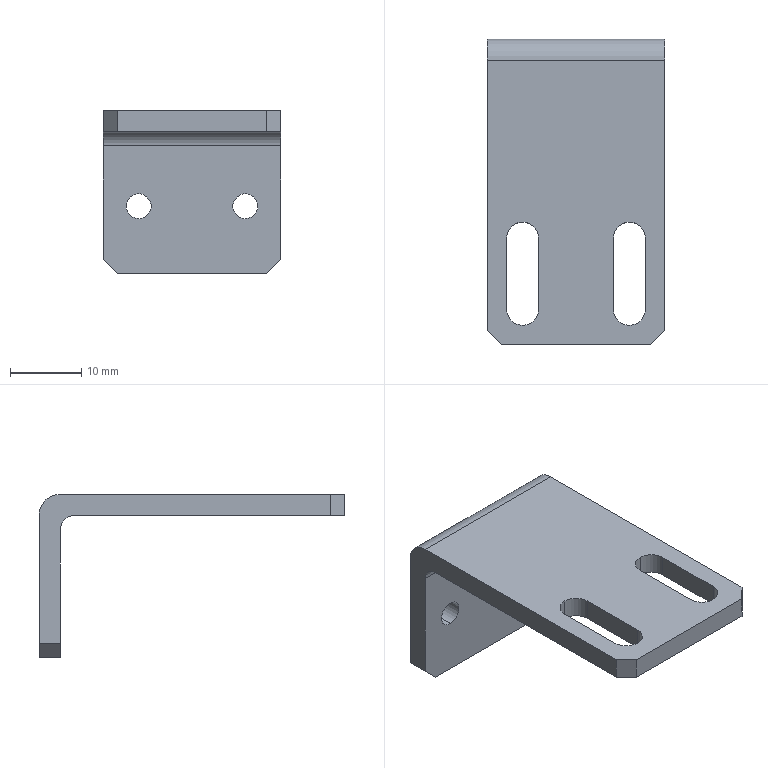Component | SolidWorks | 300-01-1 | 1 solid | 28 faces | box 25 x 43 x 23 mm | volume 4251 mm3 | plane 16 | cylinder 12 | commonest cylinder face diameters 4.5 x6 3.5 x4 6 x1 4 x1 | material SUS304
build123d program:
from build123d import *

# Parameters (mm, degrees)
EXTRUDE_THIN1_DEPTH = 12.5
CUT_EXTRUDE1_DEPTH  = 47.435
SKETCH3_R           = 1.75
CUT_EXTRUDE2_DEPTH  = 50.043
CHAMFER1_SIZE       = 2
FILLET1_R           = 3
FILLET2_R           = 2


with BuildPart() as part:
    # Sketch1 → Extrude-Thin1 (new, symmetric)
    with BuildSketch(Plane(origin=(0, 0, 0), x_dir=(1, 0, 0), z_dir=(0, 1, 0))):
        Polygon((0, 20), (0, 0), (40, 0), (40, -3), (-3, -3), (-3, 20), align=None)
    extrude(amount=EXTRUDE_THIN1_DEPTH, both=True)

    # Sketch2 → Cut-Extrude1 (cut, through all)
    with BuildSketch(Plane(origin=(0, 0, 0), x_dir=(-1, 0, 0), z_dir=(0, 0, -1))):
        with BuildLine():
            Line((-35, 9.75), (-25, 9.75))
            ThreePointArc((-25, 9.75), (-22.75, 7.5), (-25, 5.25))
            Line((-25, 5.25), (-35, 5.25))
            ThreePointArc((-35, 5.25), (-37.25, 7.5), (-35, 9.75))
        make_face()
        with BuildLine():
            Line((-35, -9.75), (-25, -9.75))
            ThreePointArc((-25, -9.75), (-22.75, -7.5), (-25, -5.25))
            Line((-25, -5.25), (-35, -5.25))
            ThreePointArc((-35, -5.25), (-37.25, -7.5), (-35, -9.75))
        make_face()
    extrude(amount=-CUT_EXTRUDE1_DEPTH, mode=Mode.SUBTRACT)

    # Sketch3 → Cut-Extrude2 (cut, through all)
    with BuildSketch(Plane.ZY.offset(3)):
        with Locations((-10.5, 7.5)):
            Circle(SKETCH3_R)
        with Locations((-10.5, -7.5)):
            Circle(SKETCH3_R)
    extrude(amount=-CUT_EXTRUDE2_DEPTH, mode=Mode.SUBTRACT)

    # Chamfer1
    chamfer1_edges = [part.edges().sort_by_distance(p)[0] for p in [
        (-1.5, 12.5, -20),
        (-1.5, -12.5, -20),
        (40, -12.5, 1.5),
        (40, 12.5, 1.5),
    ]]
    chamfer(chamfer1_edges, length=CHAMFER1_SIZE)

    # Fillet1
    fillet1_edges = [part.edges().sort_by_distance(p)[0] for p in [
        (-3, 0, 3),
    ]]
    fillet(fillet1_edges, radius=FILLET1_R)

    # Fillet2
    fillet2_edges = [part.edges().sort_by_distance(p)[0] for p in [
        (0, 0, 0),
    ]]
    fillet(fillet2_edges, radius=FILLET2_R)


solid = part.part

# Placed as in the assembly
solid = solid.moved(Location((230, 175, 115), (0, 0, -90)))
STEP:
#1=CARTESIAN_POINT('',(8.76,6.89,4.183));
#2=VERTEX_POINT('',#1);
#3=CARTESIAN_POINT('',(8.76,6.89,4.045));
#4=VERTEX_POINT('',#3);
#5=CARTESIAN_POINT('',(8.76,6.89,4.114));
#6=DIRECTION('',(-0.,-1.,0.));
#7=DIRECTION('',(0.,0.,-1.));
#8=AXIS2_PLACEMENT_3D('',#5,#6,#7);
#9=CIRCLE('',#8,0.0689);
#10=EDGE_CURVE('',#2,#4,#9,.T.);
#11=ORIENTED_EDGE('',*,*,#10,.T.);
#12=CARTESIAN_POINT('',(8.76,7.008,4.045));
#13=VERTEX_POINT('',#12);
#14=CARTESIAN_POINT('',(8.76,5.315,4.045));
#15=DIRECTION('',(0.,1.,-0.));
#16=VECTOR('',#15,39.37);
#17=LINE('',#14,#16);
#18=EDGE_CURVE('',#4,#13,#17,.T.);
#19=ORIENTED_EDGE('',*,*,#18,.T.);
#20=CARTESIAN_POINT('',(8.76,7.008,4.183));
#21=VERTEX_POINT('',#20);
#22=CARTESIAN_POINT('',(8.76,7.008,4.114));
#23=DIRECTION('',(0.,1.,-0.));
#24=DIRECTION('',(-0.,0.,1.));
#25=AXIS2_PLACEMENT_3D('',#22,#23,#24);
#26=CIRCLE('',#25,0.0689);
#27=EDGE_CURVE('',#13,#21,#26,.T.);
#28=ORIENTED_EDGE('',*,*,#27,.T.);
#29=CARTESIAN_POINT('',(8.76,5.315,4.183));
#30=DIRECTION('',(0.,1.,-0.));
#31=VECTOR('',#30,39.37);
#32=LINE('',#29,#31);
#33=EDGE_CURVE('',#2,#21,#32,.T.);
#34=ORIENTED_EDGE('',*,*,#33,.F.);
#35=EDGE_LOOP('',(#11,#19,#28,#34));
#36=FACE_OUTER_BOUND('',#35,.T.);
#37=CARTESIAN_POINT('',(8.76,5.315,4.114));
#38=DIRECTION('',(0.,1.,-0.));
#39=DIRECTION('',(-0.,0.,1.));
#40=AXIS2_PLACEMENT_3D('',#37,#38,#39);
#41=CYLINDRICAL_SURFACE('',#40,0.0689);
#42=ADVANCED_FACE('',(#36),#41,.F.);
#43=CARTESIAN_POINT('',(9.35,6.89,4.183));
#44=VERTEX_POINT('',#43);
#45=CARTESIAN_POINT('',(9.35,6.89,4.045));
#46=VERTEX_POINT('',#45);
#47=CARTESIAN_POINT('',(9.35,6.89,4.114));
#48=DIRECTION('',(-0.,-1.,0.));
#49=DIRECTION('',(0.,0.,-1.));
#50=AXIS2_PLACEMENT_3D('',#47,#48,#49);
#51=CIRCLE('',#50,0.0689);
#52=EDGE_CURVE('',#44,#46,#51,.T.);
#53=ORIENTED_EDGE('',*,*,#52,.T.);
#54=CARTESIAN_POINT('',(9.35,7.008,4.045));
#55=VERTEX_POINT('',#54);
#56=CARTESIAN_POINT('',(9.35,5.315,4.045));
#57=DIRECTION('',(0.,1.,-0.));
#58=VECTOR('',#57,39.37);
#59=LINE('',#56,#58);
#60=EDGE_CURVE('',#46,#55,#59,.T.);
#61=ORIENTED_EDGE('',*,*,#60,.T.);
#62=CARTESIAN_POINT('',(9.35,7.008,4.183));
#63=VERTEX_POINT('',#62);
#64=CARTESIAN_POINT('',(9.35,7.008,4.114));
#65=DIRECTION('',(0.,1.,-0.));
#66=DIRECTION('',(-0.,0.,1.));
#67=AXIS2_PLACEMENT_3D('',#64,#65,#66);
#68=CIRCLE('',#67,0.0689);
#69=EDGE_CURVE('',#55,#63,#68,.T.);
#70=ORIENTED_EDGE('',*,*,#69,.T.);
#71=CARTESIAN_POINT('',(9.35,5.315,4.183));
#72=DIRECTION('',(0.,1.,-0.));
#73=VECTOR('',#72,39.37);
#74=LINE('',#71,#73);
#75=EDGE_CURVE('',#44,#63,#74,.T.);
#76=ORIENTED_EDGE('',*,*,#75,.F.);
#77=EDGE_LOOP('',(#53,#61,#70,#76));
#78=FACE_OUTER_BOUND('',#77,.T.);
#79=CARTESIAN_POINT('',(9.35,5.315,4.114));
#80=DIRECTION('',(0.,1.,-0.));
#81=DIRECTION('',(-0.,0.,1.));
#82=AXIS2_PLACEMENT_3D('',#79,#80,#81);
#83=CYLINDRICAL_SURFACE('',#82,0.0689);
#84=ADVANCED_FACE('',(#78),#83,.F.);
#85=CARTESIAN_POINT('',(8.76,5.994,4.646));
#86=VERTEX_POINT('',#85);
#87=CARTESIAN_POINT('',(8.848,5.906,4.646));
#88=VERTEX_POINT('',#87);
#89=CARTESIAN_POINT('',(8.76,5.906,4.646));
#90=DIRECTION('',(0.,-0.,-1.));
#91=DIRECTION('',(0.,-1.,0.));
#92=AXIS2_PLACEMENT_3D('',#89,#90,#91);
#93=CIRCLE('',#92,0.08858);
#94=EDGE_CURVE('',#86,#88,#93,.T.);
#95=ORIENTED_EDGE('',*,*,#94,.F.);
#96=CARTESIAN_POINT('',(8.76,5.994,4.528));
#97=VERTEX_POINT('',#96);
#98=CARTESIAN_POINT('',(8.76,5.994,4.646));
#99=DIRECTION('',(0.,-0.,-1.));
#100=VECTOR('',#99,39.37);
#101=LINE('',#98,#100);
#102=EDGE_CURVE('',#86,#97,#101,.T.);
#103=ORIENTED_EDGE('',*,*,#102,.T.);
#104=CARTESIAN_POINT('',(8.848,5.906,4.528));
#105=VERTEX_POINT('',#104);
#106=CARTESIAN_POINT('',(8.76,5.906,4.528));
#107=DIRECTION('',(0.,-0.,-1.));
#108=DIRECTION('',(0.,-1.,0.));
#109=AXIS2_PLACEMENT_3D('',#106,#107,#108);
#110=CIRCLE('',#109,0.08858);
#111=EDGE_CURVE('',#97,#105,#110,.T.);
#112=ORIENTED_EDGE('',*,*,#111,.T.);
#113=CARTESIAN_POINT('',(8.848,5.906,4.646));
#114=DIRECTION('',(0.,-0.,-1.));
#115=VECTOR('',#114,39.37);
#116=LINE('',#113,#115);
#117=EDGE_CURVE('',#88,#105,#116,.T.);
#118=ORIENTED_EDGE('',*,*,#117,.F.);
#119=EDGE_LOOP('',(#95,#103,#112,#118));
#120=FACE_OUTER_BOUND('',#119,.T.);
#121=CARTESIAN_POINT('',(8.76,5.906,4.646));
#122=DIRECTION('',(0.,-0.,-1.));
#123=DIRECTION('',(0.,1.,0.));
#124=AXIS2_PLACEMENT_3D('',#121,#122,#123);
#125=CYLINDRICAL_SURFACE('',#124,0.08858);
#126=ADVANCED_FACE('',(#120),#125,.F.);
#127=CARTESIAN_POINT('',(9.35,5.994,4.646));
#128=VERTEX_POINT('',#127);
#129=CARTESIAN_POINT('',(9.439,5.906,4.646));
#130=VERTEX_POINT('',#129);
#131=CARTESIAN_POINT('',(9.35,5.906,4.646));
#132=DIRECTION('',(0.,-0.,-1.));
#133=DIRECTION('',(0.,1.,0.));
#134=AXIS2_PLACEMENT_3D('',#131,#132,#133);
#135=CIRCLE('',#134,0.08858);
#136=EDGE_CURVE('',#128,#130,#135,.T.);
#137=ORIENTED_EDGE('',*,*,#136,.F.);
#138=CARTESIAN_POINT('',(9.35,5.994,4.528));
#139=VERTEX_POINT('',#138);
#140=CARTESIAN_POINT('',(9.35,5.994,4.646));
#141=DIRECTION('',(0.,-0.,-1.));
#142=VECTOR('',#141,39.37);
#143=LINE('',#140,#142);
#144=EDGE_CURVE('',#128,#139,#143,.T.);
#145=ORIENTED_EDGE('',*,*,#144,.T.);
#146=CARTESIAN_POINT('',(9.439,5.906,4.528));
#147=VERTEX_POINT('',#146);
#148=CARTESIAN_POINT('',(9.35,5.906,4.528));
#149=DIRECTION('',(0.,-0.,-1.));
#150=DIRECTION('',(0.,1.,0.));
#151=AXIS2_PLACEMENT_3D('',#148,#149,#150);
#152=CIRCLE('',#151,0.08858);
#153=EDGE_CURVE('',#139,#147,#152,.T.);
#154=ORIENTED_EDGE('',*,*,#153,.T.);
#155=CARTESIAN_POINT('',(9.439,5.906,4.646));
#156=DIRECTION('',(0.,-0.,-1.));
#157=VECTOR('',#156,39.37);
#158=LINE('',#155,#157);
#159=EDGE_CURVE('',#130,#147,#158,.T.);
#160=ORIENTED_EDGE('',*,*,#159,.F.);
#161=EDGE_LOOP('',(#137,#145,#154,#160));
#162=FACE_OUTER_BOUND('',#161,.T.);
#163=CARTESIAN_POINT('',(9.35,5.906,4.646));
#164=DIRECTION('',(0.,-0.,-1.));
#165=DIRECTION('',(0.,1.,0.));
#166=AXIS2_PLACEMENT_3D('',#163,#164,#165);
#167=CYLINDRICAL_SURFACE('',#166,0.08858);
#168=ADVANCED_FACE('',(#162),#167,.F.);
#169=CARTESIAN_POINT('',(8.848,5.512,4.646));
#170=VERTEX_POINT('',#169);
#171=CARTESIAN_POINT('',(8.848,5.512,4.646));
#172=DIRECTION('',(-0.,-1.,0.));
#173=VECTOR('',#172,39.37);
#174=LINE('',#171,#173);
#175=EDGE_CURVE('',#88,#170,#174,.T.);
#176=ORIENTED_EDGE('',*,*,#175,.T.);
#177=CARTESIAN_POINT('',(8.671,5.512,4.646));
#178=VERTEX_POINT('',#177);
#179=CARTESIAN_POINT('',(8.76,5.512,4.646));
#180=DIRECTION('',(0.,-0.,-1.));
#181=DIRECTION('',(0.,-1.,0.));
#182=AXIS2_PLACEMENT_3D('',#179,#180,#181);
#183=CIRCLE('',#182,0.08858);
#184=EDGE_CURVE('',#170,#178,#183,.T.);
#185=ORIENTED_EDGE('',*,*,#184,.T.);
#186=CARTESIAN_POINT('',(8.671,5.906,4.646));
#187=VERTEX_POINT('',#186);
#188=CARTESIAN_POINT('',(8.671,5.512,4.646));
#189=DIRECTION('',(0.,1.,-0.));
#190=VECTOR('',#189,39.37);
#191=LINE('',#188,#190);
#192=EDGE_CURVE('',#178,#187,#191,.T.);
#193=ORIENTED_EDGE('',*,*,#192,.T.);
#194=CARTESIAN_POINT('',(8.76,5.906,4.646));
#195=DIRECTION('',(0.,-0.,-1.));
#196=DIRECTION('',(0.,-1.,0.));
#197=AXIS2_PLACEMENT_3D('',#194,#195,#196);
#198=CIRCLE('',#197,0.08858);
#199=EDGE_CURVE('',#187,#86,#198,.T.);
#200=ORIENTED_EDGE('',*,*,#199,.T.);
#201=ORIENTED_EDGE('',*,*,#94,.T.);
#202=EDGE_LOOP('',(#176,#185,#193,#200,#201));
#203=FACE_BOUND('',#202,.T.);
#204=CARTESIAN_POINT('',(9.439,5.512,4.646));
#205=VERTEX_POINT('',#204);
#206=CARTESIAN_POINT('',(9.439,5.512,4.646));
#207=DIRECTION('',(0.,-1.,0.));
#208=VECTOR('',#207,39.37);
#209=LINE('',#206,#208);
#210=EDGE_CURVE('',#130,#205,#209,.T.);
#211=ORIENTED_EDGE('',*,*,#210,.T.);
#212=CARTESIAN_POINT('',(9.262,5.512,4.646));
#213=VERTEX_POINT('',#212);
#214=CARTESIAN_POINT('',(9.35,5.512,4.646));
#215=DIRECTION('',(0.,-0.,-1.));
#216=DIRECTION('',(0.,1.,0.));
#217=AXIS2_PLACEMENT_3D('',#214,#215,#216);
#218=CIRCLE('',#217,0.08858);
#219=EDGE_CURVE('',#205,#213,#218,.T.);
#220=ORIENTED_EDGE('',*,*,#219,.T.);
#221=CARTESIAN_POINT('',(9.262,5.906,4.646));
#222=VERTEX_POINT('',#221);
#223=CARTESIAN_POINT('',(9.262,5.512,4.646));
#224=DIRECTION('',(0.,1.,-0.));
#225=VECTOR('',#224,39.37);
#226=LINE('',#223,#225);
#227=EDGE_CURVE('',#213,#222,#226,.T.);
#228=ORIENTED_EDGE('',*,*,#227,.T.);
#229=CARTESIAN_POINT('',(9.35,5.906,4.646));
#230=DIRECTION('',(0.,-0.,-1.));
#231=DIRECTION('',(0.,1.,0.));
#232=AXIS2_PLACEMENT_3D('',#229,#230,#231);
#233=CIRCLE('',#232,0.08858);
#234=EDGE_CURVE('',#222,#128,#233,.T.);
#235=ORIENTED_EDGE('',*,*,#234,.T.);
#236=ORIENTED_EDGE('',*,*,#136,.T.);
#237=EDGE_LOOP('',(#211,#220,#228,#235,#236));
#238=FACE_BOUND('',#237,.T.);
#239=CARTESIAN_POINT('',(9.547,6.89,4.646));
#240=VERTEX_POINT('',#239);
#241=CARTESIAN_POINT('',(9.547,5.394,4.646));
#242=VERTEX_POINT('',#241);
#243=CARTESIAN_POINT('',(9.547,6.89,4.646));
#244=DIRECTION('',(-0.,-1.,0.));
#245=VECTOR('',#244,39.37);
#246=LINE('',#243,#245);
#247=EDGE_CURVE('',#240,#242,#246,.T.);
#248=ORIENTED_EDGE('',*,*,#247,.F.);
#249=CARTESIAN_POINT('',(8.563,6.89,4.646));
#250=VERTEX_POINT('',#249);
#251=CARTESIAN_POINT('',(9.547,6.89,4.646));
#252=DIRECTION('',(-1.,0.,-0.));
#253=VECTOR('',#252,39.37);
#254=LINE('',#251,#253);
#255=EDGE_CURVE('',#240,#250,#254,.T.);
#256=ORIENTED_EDGE('',*,*,#255,.T.);
#257=CARTESIAN_POINT('',(8.563,5.394,4.646));
#258=VERTEX_POINT('',#257);
#259=CARTESIAN_POINT('',(8.563,6.89,4.646));
#260=DIRECTION('',(-0.,-1.,0.));
#261=VECTOR('',#260,39.37);
#262=LINE('',#259,#261);
#263=EDGE_CURVE('',#250,#258,#262,.T.);
#264=ORIENTED_EDGE('',*,*,#263,.T.);
#265=CARTESIAN_POINT('',(8.642,5.315,4.646));
#266=VERTEX_POINT('',#265);
#267=CARTESIAN_POINT('',(8.563,5.394,4.646));
#268=DIRECTION('',(0.7071,-0.7071,0.));
#269=VECTOR('',#268,39.37);
#270=LINE('',#267,#269);
#271=EDGE_CURVE('',#258,#266,#270,.T.);
#272=ORIENTED_EDGE('',*,*,#271,.T.);
#273=CARTESIAN_POINT('',(9.469,5.315,4.646));
#274=VERTEX_POINT('',#273);
#275=CARTESIAN_POINT('',(9.547,5.315,4.646));
#276=DIRECTION('',(-1.,0.,-0.));
#277=VECTOR('',#276,39.37);
#278=LINE('',#275,#277);
#279=EDGE_CURVE('',#274,#266,#278,.T.);
#280=ORIENTED_EDGE('',*,*,#279,.F.);
#281=CARTESIAN_POINT('',(9.469,5.315,4.646));
#282=DIRECTION('',(0.7071,0.7071,0.));
#283=VECTOR('',#282,39.37);
#284=LINE('',#281,#283);
#285=EDGE_CURVE('',#274,#242,#284,.T.);
#286=ORIENTED_EDGE('',*,*,#285,.T.);
#287=EDGE_LOOP('',(#248,#256,#264,#272,#280,#286));
#288=FACE_OUTER_BOUND('',#287,.T.);
#289=CARTESIAN_POINT('',(9.547,6.89,4.646));
#290=DIRECTION('',(0.,-0.,-1.));
#291=DIRECTION('',(0.,1.,-0.));
#292=AXIS2_PLACEMENT_3D('',#289,#290,#291);
#293=PLANE('',#292);
#294=ADVANCED_FACE('',(#203,#238,#288),#293,.F.);
#295=CARTESIAN_POINT('',(9.469,5.315,4.528));
#296=VERTEX_POINT('',#295);
#297=CARTESIAN_POINT('',(8.642,5.315,4.528));
#298=VERTEX_POINT('',#297);
#299=CARTESIAN_POINT('',(9.547,5.315,4.528));
#300=DIRECTION('',(-1.,0.,-0.));
#301=VECTOR('',#300,39.37);
#302=LINE('',#299,#301);
#303=EDGE_CURVE('',#296,#298,#302,.T.);
#304=ORIENTED_EDGE('',*,*,#303,.F.);
#305=CARTESIAN_POINT('',(9.469,5.315,4.646));
#306=DIRECTION('',(-0.,0.,1.));
#307=VECTOR('',#306,39.37);
#308=LINE('',#305,#307);
#309=EDGE_CURVE('',#296,#274,#308,.T.);
#310=ORIENTED_EDGE('',*,*,#309,.T.);
#311=ORIENTED_EDGE('',*,*,#279,.T.);
#312=CARTESIAN_POINT('',(8.642,5.315,4.528));
#313=DIRECTION('',(0.,-0.,-1.));
#314=VECTOR('',#313,39.37);
#315=LINE('',#312,#314);
#316=EDGE_CURVE('',#266,#298,#315,.T.);
#317=ORIENTED_EDGE('',*,*,#316,.T.);
#318=EDGE_LOOP('',(#304,#310,#311,#317));
#319=FACE_OUTER_BOUND('',#318,.T.);
#320=CARTESIAN_POINT('',(9.547,5.315,4.528));
#321=DIRECTION('',(-0.,-1.,0.));
#322=DIRECTION('',(0.,-0.,-1.));
#323=AXIS2_PLACEMENT_3D('',#320,#321,#322);
#324=PLANE('',#323);
#325=ADVANCED_FACE('',(#319),#324,.T.);
#326=CARTESIAN_POINT('',(8.848,5.512,4.528));
#327=VERTEX_POINT('',#326);
#328=CARTESIAN_POINT('',(8.671,5.512,4.528));
#329=VERTEX_POINT('',#328);
#330=CARTESIAN_POINT('',(8.76,5.512,4.528));
#331=DIRECTION('',(0.,-0.,-1.));
#332=DIRECTION('',(0.,-1.,0.));
#333=AXIS2_PLACEMENT_3D('',#330,#331,#332);
#334=CIRCLE('',#333,0.08858);
#335=EDGE_CURVE('',#327,#329,#334,.T.);
#336=ORIENTED_EDGE('',*,*,#335,.F.);
#337=CARTESIAN_POINT('',(8.848,5.512,4.528));
#338=DIRECTION('',(-0.,-1.,0.));
#339=VECTOR('',#338,39.37);
#340=LINE('',#337,#339);
#341=EDGE_CURVE('',#105,#327,#340,.T.);
#342=ORIENTED_EDGE('',*,*,#341,.F.);
#343=ORIENTED_EDGE('',*,*,#111,.F.);
#344=CARTESIAN_POINT('',(8.671,5.906,4.528));
#345=VERTEX_POINT('',#344);
#346=CARTESIAN_POINT('',(8.76,5.906,4.528));
#347=DIRECTION('',(0.,-0.,-1.));
#348=DIRECTION('',(0.,-1.,0.));
#349=AXIS2_PLACEMENT_3D('',#346,#347,#348);
#350=CIRCLE('',#349,0.08858);
#351=EDGE_CURVE('',#345,#97,#350,.T.);
#352=ORIENTED_EDGE('',*,*,#351,.F.);
#353=CARTESIAN_POINT('',(8.671,5.512,4.528));
#354=DIRECTION('',(0.,1.,-0.));
#355=VECTOR('',#354,39.37);
#356=LINE('',#353,#355);
#357=EDGE_CURVE('',#329,#345,#356,.T.);
#358=ORIENTED_EDGE('',*,*,#357,.F.);
#359=EDGE_LOOP('',(#336,#342,#343,#352,#358));
#360=FACE_BOUND('',#359,.T.);
#361=CARTESIAN_POINT('',(9.439,5.512,4.528));
#362=VERTEX_POINT('',#361);
#363=CARTESIAN_POINT('',(9.262,5.512,4.528));
#364=VERTEX_POINT('',#363);
#365=CARTESIAN_POINT('',(9.35,5.512,4.528));
#366=DIRECTION('',(0.,-0.,-1.));
#367=DIRECTION('',(0.,1.,0.));
#368=AXIS2_PLACEMENT_3D('',#365,#366,#367);
#369=CIRCLE('',#368,0.08858);
#370=EDGE_CURVE('',#362,#364,#369,.T.);
#371=ORIENTED_EDGE('',*,*,#370,.F.);
#372=CARTESIAN_POINT('',(9.439,5.512,4.528));
#373=DIRECTION('',(0.,-1.,0.));
#374=VECTOR('',#373,39.37);
#375=LINE('',#372,#374);
#376=EDGE_CURVE('',#147,#362,#375,.T.);
#377=ORIENTED_EDGE('',*,*,#376,.F.);
#378=ORIENTED_EDGE('',*,*,#153,.F.);
#379=CARTESIAN_POINT('',(9.262,5.906,4.528));
#380=VERTEX_POINT('',#379);
#381=CARTESIAN_POINT('',(9.35,5.906,4.528));
#382=DIRECTION('',(0.,-0.,-1.));
#383=DIRECTION('',(0.,1.,0.));
#384=AXIS2_PLACEMENT_3D('',#381,#382,#383);
#385=CIRCLE('',#384,0.08858);
#386=EDGE_CURVE('',#380,#139,#385,.T.);
#387=ORIENTED_EDGE('',*,*,#386,.F.);
#388=CARTESIAN_POINT('',(9.262,5.512,4.528));
#389=DIRECTION('',(0.,1.,-0.));
#390=VECTOR('',#389,39.37);
#391=LINE('',#388,#390);
#392=EDGE_CURVE('',#364,#380,#391,.T.);
#393=ORIENTED_EDGE('',*,*,#392,.F.);
#394=EDGE_LOOP('',(#371,#377,#378,#387,#393));
#395=FACE_BOUND('',#394,.T.);
#396=CARTESIAN_POINT('',(8.563,6.811,4.528));
#397=VERTEX_POINT('',#396);
#398=CARTESIAN_POINT('',(8.563,5.394,4.528));
#399=VERTEX_POINT('',#398);
#400=CARTESIAN_POINT('',(8.563,6.89,4.528));
#401=DIRECTION('',(-0.,-1.,0.));
#402=VECTOR('',#401,39.37);
#403=LINE('',#400,#402);
#404=EDGE_CURVE('',#397,#399,#403,.T.);
#405=ORIENTED_EDGE('',*,*,#404,.F.);
#406=CARTESIAN_POINT('',(9.547,6.811,4.528));
#407=VERTEX_POINT('',#406);
#408=CARTESIAN_POINT('',(9.547,6.811,4.528));
#409=DIRECTION('',(1.,-0.,0.));
#410=VECTOR('',#409,39.37);
#411=LINE('',#408,#410);
#412=EDGE_CURVE('',#397,#407,#411,.T.);
#413=ORIENTED_EDGE('',*,*,#412,.T.);
#414=CARTESIAN_POINT('',(9.547,5.394,4.528));
#415=VERTEX_POINT('',#414);
#416=CARTESIAN_POINT('',(9.547,6.89,4.528));
#417=DIRECTION('',(-0.,-1.,0.));
#418=VECTOR('',#417,39.37);
#419=LINE('',#416,#418);
#420=EDGE_CURVE('',#407,#415,#419,.T.);
#421=ORIENTED_EDGE('',*,*,#420,.T.);
#422=CARTESIAN_POINT('',(10.295,6.142,4.528));
#423=DIRECTION('',(-0.7071,-0.7071,-0.));
#424=VECTOR('',#423,39.37);
#425=LINE('',#422,#424);
#426=EDGE_CURVE('',#415,#296,#425,.T.);
#427=ORIENTED_EDGE('',*,*,#426,.T.);
#428=ORIENTED_EDGE('',*,*,#303,.T.);
#429=CARTESIAN_POINT('',(8.307,5.65,4.528));
#430=DIRECTION('',(-0.7071,0.7071,-0.));
#431=VECTOR('',#430,39.37);
#432=LINE('',#429,#431);
#433=EDGE_CURVE('',#298,#399,#432,.T.);
#434=ORIENTED_EDGE('',*,*,#433,.T.);
#435=EDGE_LOOP('',(#405,#413,#421,#427,#428,#434));
#436=FACE_OUTER_BOUND('',#435,.T.);
#437=CARTESIAN_POINT('',(9.547,6.89,4.528));
#438=DIRECTION('',(0.,-0.,-1.));
#439=DIRECTION('',(0.,1.,-0.));
#440=AXIS2_PLACEMENT_3D('',#437,#438,#439);
#441=PLANE('',#440);
#442=ADVANCED_FACE('',(#360,#395,#436),#441,.T.);
#443=ORIENTED_EDGE('',*,*,#10,.F.);
#444=CARTESIAN_POINT('',(8.76,6.89,4.114));
#445=DIRECTION('',(-0.,-1.,0.));
#446=DIRECTION('',(0.,0.,-1.));
#447=AXIS2_PLACEMENT_3D('',#444,#445,#446);
#448=CIRCLE('',#447,0.0689);
#449=EDGE_CURVE('',#4,#2,#448,.T.);
#450=ORIENTED_EDGE('',*,*,#449,.F.);
#451=EDGE_LOOP('',(#443,#450));
#452=FACE_BOUND('',#451,.T.);
#453=ORIENTED_EDGE('',*,*,#52,.F.);
#454=CARTESIAN_POINT('',(9.35,6.89,4.114));
#455=DIRECTION('',(-0.,-1.,0.));
#456=DIRECTION('',(0.,0.,-1.));
#457=AXIS2_PLACEMENT_3D('',#454,#455,#456);
#458=CIRCLE('',#457,0.0689);
#459=EDGE_CURVE('',#46,#44,#458,.T.);
#460=ORIENTED_EDGE('',*,*,#459,.F.);
#461=EDGE_LOOP('',(#453,#460));
#462=FACE_BOUND('',#461,.T.);
#463=CARTESIAN_POINT('',(9.547,6.89,3.819));
#464=VERTEX_POINT('',#463);
#465=CARTESIAN_POINT('',(9.547,6.89,4.449));
#466=VERTEX_POINT('',#465);
#467=CARTESIAN_POINT('',(9.547,6.89,3.74));
#468=DIRECTION('',(-0.,0.,1.));
#469=VECTOR('',#468,39.37);
#470=LINE('',#467,#469);
#471=EDGE_CURVE('',#464,#466,#470,.T.);
#472=ORIENTED_EDGE('',*,*,#471,.T.);
#473=CARTESIAN_POINT('',(8.563,6.89,4.449));
#474=VERTEX_POINT('',#473);
#475=CARTESIAN_POINT('',(8.563,6.89,4.449));
#476=DIRECTION('',(-1.,0.,-0.));
#477=VECTOR('',#476,39.37);
#478=LINE('',#475,#477);
#479=EDGE_CURVE('',#466,#474,#478,.T.);
#480=ORIENTED_EDGE('',*,*,#479,.T.);
#481=CARTESIAN_POINT('',(8.563,6.89,3.819));
#482=VERTEX_POINT('',#481);
#483=CARTESIAN_POINT('',(8.563,6.89,3.74));
#484=DIRECTION('',(-0.,0.,1.));
#485=VECTOR('',#484,39.37);
#486=LINE('',#483,#485);
#487=EDGE_CURVE('',#482,#474,#486,.T.);
#488=ORIENTED_EDGE('',*,*,#487,.F.);
#489=CARTESIAN_POINT('',(8.642,6.89,3.74));
#490=VERTEX_POINT('',#489);
#491=CARTESIAN_POINT('',(9.094,6.89,3.287));
#492=DIRECTION('',(0.7071,-0.,-0.7071));
#493=VECTOR('',#492,39.37);
#494=LINE('',#491,#493);
#495=EDGE_CURVE('',#482,#490,#494,.T.);
#496=ORIENTED_EDGE('',*,*,#495,.T.);
#497=CARTESIAN_POINT('',(9.469,6.89,3.74));
#498=VERTEX_POINT('',#497);
#499=CARTESIAN_POINT('',(9.547,6.89,3.74));
#500=DIRECTION('',(-1.,0.,-0.));
#501=VECTOR('',#500,39.37);
#502=LINE('',#499,#501);
#503=EDGE_CURVE('',#498,#490,#502,.T.);
#504=ORIENTED_EDGE('',*,*,#503,.F.);
#505=CARTESIAN_POINT('',(9.508,6.89,3.78));
#506=DIRECTION('',(0.7071,0.,0.7071));
#507=VECTOR('',#506,39.37);
#508=LINE('',#505,#507);
#509=EDGE_CURVE('',#498,#464,#508,.T.);
#510=ORIENTED_EDGE('',*,*,#509,.T.);
#511=EDGE_LOOP('',(#472,#480,#488,#496,#504,#510));
#512=FACE_OUTER_BOUND('',#511,.T.);
#513=CARTESIAN_POINT('',(9.547,6.89,3.74));
#514=DIRECTION('',(-0.,-1.,0.));
#515=DIRECTION('',(0.,-0.,-1.));
#516=AXIS2_PLACEMENT_3D('',#513,#514,#515);
#517=PLANE('',#516);
#518=ADVANCED_FACE('',(#452,#462,#512),#517,.T.);
#519=ORIENTED_EDGE('',*,*,#503,.T.);
#520=CARTESIAN_POINT('',(8.642,7.008,3.74));
#521=VERTEX_POINT('',#520);
#522=CARTESIAN_POINT('',(8.642,7.008,3.74));
#523=DIRECTION('',(0.,1.,-0.));
#524=VECTOR('',#523,39.37);
#525=LINE('',#522,#524);
#526=EDGE_CURVE('',#490,#521,#525,.T.);
#527=ORIENTED_EDGE('',*,*,#526,.T.);
#528=CARTESIAN_POINT('',(9.469,7.008,3.74));
#529=VERTEX_POINT('',#528);
#530=CARTESIAN_POINT('',(9.547,7.008,3.74));
#531=DIRECTION('',(-1.,0.,-0.));
#532=VECTOR('',#531,39.37);
#533=LINE('',#530,#532);
#534=EDGE_CURVE('',#529,#521,#533,.T.);
#535=ORIENTED_EDGE('',*,*,#534,.F.);
#536=CARTESIAN_POINT('',(9.469,6.89,3.74));
#537=DIRECTION('',(-0.,-1.,0.));
#538=VECTOR('',#537,39.37);
#539=LINE('',#536,#538);
#540=EDGE_CURVE('',#529,#498,#539,.T.);
#541=ORIENTED_EDGE('',*,*,#540,.T.);
#542=EDGE_LOOP('',(#519,#527,#535,#541));
#543=FACE_OUTER_BOUND('',#542,.T.);
#544=CARTESIAN_POINT('',(9.547,7.008,3.74));
#545=DIRECTION('',(0.,-0.,-1.));
#546=DIRECTION('',(0.,1.,-0.));
#547=AXIS2_PLACEMENT_3D('',#544,#545,#546);
#548=PLANE('',#547);
#549=ADVANCED_FACE('',(#543),#548,.T.);
#550=CARTESIAN_POINT('',(8.76,7.008,4.114));
#551=DIRECTION('',(0.,1.,-0.));
#552=DIRECTION('',(-0.,0.,1.));
#553=AXIS2_PLACEMENT_3D('',#550,#551,#552);
#554=CIRCLE('',#553,0.0689);
#555=EDGE_CURVE('',#21,#13,#554,.T.);
#556=ORIENTED_EDGE('',*,*,#555,.F.);
#557=ORIENTED_EDGE('',*,*,#27,.F.);
#558=EDGE_LOOP('',(#556,#557));
#559=FACE_BOUND('',#558,.T.);
#560=CARTESIAN_POINT('',(9.35,7.008,4.114));
#561=DIRECTION('',(0.,1.,-0.));
#562=DIRECTION('',(-0.,0.,1.));
#563=AXIS2_PLACEMENT_3D('',#560,#561,#562);
#564=CIRCLE('',#563,0.0689);
#565=EDGE_CURVE('',#63,#55,#564,.T.);
#566=ORIENTED_EDGE('',*,*,#565,.F.);
#567=ORIENTED_EDGE('',*,*,#69,.F.);
#568=EDGE_LOOP('',(#566,#567));
#569=FACE_BOUND('',#568,.T.);
#570=CARTESIAN_POINT('',(8.563,7.008,3.819));
#571=VERTEX_POINT('',#570);
#572=CARTESIAN_POINT('',(8.563,7.008,4.528));
#573=VERTEX_POINT('',#572);
#574=CARTESIAN_POINT('',(8.563,7.008,3.74));
#575=DIRECTION('',(-0.,0.,1.));
#576=VECTOR('',#575,39.37);
#577=LINE('',#574,#576);
#578=EDGE_CURVE('',#571,#573,#577,.T.);
#579=ORIENTED_EDGE('',*,*,#578,.T.);
#580=CARTESIAN_POINT('',(9.547,7.008,4.528));
#581=VERTEX_POINT('',#580);
#582=CARTESIAN_POINT('',(9.547,7.008,4.528));
#583=DIRECTION('',(1.,-0.,0.));
#584=VECTOR('',#583,39.37);
#585=LINE('',#582,#584);
#586=EDGE_CURVE('',#573,#581,#585,.T.);
#587=ORIENTED_EDGE('',*,*,#586,.T.);
#588=CARTESIAN_POINT('',(9.547,7.008,3.819));
#589=VERTEX_POINT('',#588);
#590=CARTESIAN_POINT('',(9.547,7.008,3.74));
#591=DIRECTION('',(-0.,0.,1.));
#592=VECTOR('',#591,39.37);
#593=LINE('',#590,#592);
#594=EDGE_CURVE('',#589,#581,#593,.T.);
#595=ORIENTED_EDGE('',*,*,#594,.F.);
#596=CARTESIAN_POINT('',(9.469,7.008,3.74));
#597=DIRECTION('',(-0.7071,-0.,-0.7071));
#598=VECTOR('',#597,39.37);
#599=LINE('',#596,#598);
#600=EDGE_CURVE('',#589,#529,#599,.T.);
#601=ORIENTED_EDGE('',*,*,#600,.T.);
#602=ORIENTED_EDGE('',*,*,#534,.T.);
#603=CARTESIAN_POINT('',(8.563,7.008,3.819));
#604=DIRECTION('',(-0.7071,0.,0.7071));
#605=VECTOR('',#604,39.37);
#606=LINE('',#603,#605);
#607=EDGE_CURVE('',#521,#571,#606,.T.);
#608=ORIENTED_EDGE('',*,*,#607,.T.);
#609=EDGE_LOOP('',(#579,#587,#595,#601,#602,#608));
#610=FACE_OUTER_BOUND('',#609,.T.);
#611=CARTESIAN_POINT('',(9.547,7.008,3.74));
#612=DIRECTION('',(-0.,-1.,0.));
#613=DIRECTION('',(0.,-0.,-1.));
#614=AXIS2_PLACEMENT_3D('',#611,#612,#613);
#615=PLANE('',#614);
#616=ADVANCED_FACE('',(#559,#569,#610),#615,.F.);
#617=ORIENTED_EDGE('',*,*,#594,.T.);
#618=CARTESIAN_POINT('',(9.547,6.89,4.528));
#619=DIRECTION('',(1.,-0.,0.));
#620=DIRECTION('',(0.,0.,-1.));
#621=AXIS2_PLACEMENT_3D('',#618,#619,#620);
#622=CIRCLE('',#621,0.1181);
#623=EDGE_CURVE('',#581,#240,#622,.T.);
#624=ORIENTED_EDGE('',*,*,#623,.T.);
#625=ORIENTED_EDGE('',*,*,#247,.T.);
#626=CARTESIAN_POINT('',(9.547,5.394,4.528));
#627=DIRECTION('',(0.,-0.,-1.));
#628=VECTOR('',#627,39.37);
#629=LINE('',#626,#628);
#630=EDGE_CURVE('',#242,#415,#629,.T.);
#631=ORIENTED_EDGE('',*,*,#630,.T.);
#632=ORIENTED_EDGE('',*,*,#420,.F.);
#633=CARTESIAN_POINT('',(9.547,6.811,4.449));
#634=DIRECTION('',(-1.,0.,-0.));
#635=DIRECTION('',(0.,0.,-1.));
#636=AXIS2_PLACEMENT_3D('',#633,#634,#635);
#637=CIRCLE('',#636,0.07874);
#638=EDGE_CURVE('',#407,#466,#637,.T.);
#639=ORIENTED_EDGE('',*,*,#638,.T.);
#640=ORIENTED_EDGE('',*,*,#471,.F.);
#641=CARTESIAN_POINT('',(9.547,7.008,3.819));
#642=DIRECTION('',(0.,1.,-0.));
#643=VECTOR('',#642,39.37);
#644=LINE('',#641,#643);
#645=EDGE_CURVE('',#464,#589,#644,.T.);
#646=ORIENTED_EDGE('',*,*,#645,.T.);
#647=EDGE_LOOP('',(#617,#624,#625,#631,#632,#639,#640,#646));
#648=FACE_OUTER_BOUND('',#647,.T.);
#649=CARTESIAN_POINT('',(9.547,6.89,4.528));
#650=DIRECTION('',(-1.,0.,-0.));
#651=DIRECTION('',(0.,1.,-0.));
#652=AXIS2_PLACEMENT_3D('',#649,#650,#651);
#653=PLANE('',#652);
#654=ADVANCED_FACE('',(#648),#653,.F.);
#655=ORIENTED_EDGE('',*,*,#263,.F.);
#656=CARTESIAN_POINT('',(8.563,6.89,4.528));
#657=DIRECTION('',(-1.,0.,-0.));
#658=DIRECTION('',(0.,0.,-1.));
#659=AXIS2_PLACEMENT_3D('',#656,#657,#658);
#660=CIRCLE('',#659,0.1181);
#661=EDGE_CURVE('',#250,#573,#660,.T.);
#662=ORIENTED_EDGE('',*,*,#661,.T.);
#663=ORIENTED_EDGE('',*,*,#578,.F.);
#664=CARTESIAN_POINT('',(8.563,6.89,3.819));
#665=DIRECTION('',(-0.,-1.,0.));
#666=VECTOR('',#665,39.37);
#667=LINE('',#664,#666);
#668=EDGE_CURVE('',#571,#482,#667,.T.);
#669=ORIENTED_EDGE('',*,*,#668,.T.);
#670=ORIENTED_EDGE('',*,*,#487,.T.);
#671=CARTESIAN_POINT('',(8.563,6.811,4.449));
#672=DIRECTION('',(1.,-0.,0.));
#673=DIRECTION('',(0.,0.,-1.));
#674=AXIS2_PLACEMENT_3D('',#671,#672,#673);
#675=CIRCLE('',#674,0.07874);
#676=EDGE_CURVE('',#474,#397,#675,.T.);
#677=ORIENTED_EDGE('',*,*,#676,.T.);
#678=ORIENTED_EDGE('',*,*,#404,.T.);
#679=CARTESIAN_POINT('',(8.563,5.394,4.528));
#680=DIRECTION('',(-0.,0.,1.));
#681=VECTOR('',#680,39.37);
#682=LINE('',#679,#681);
#683=EDGE_CURVE('',#399,#258,#682,.T.);
#684=ORIENTED_EDGE('',*,*,#683,.T.);
#685=EDGE_LOOP('',(#655,#662,#663,#669,#670,#677,#678,#684));
#686=FACE_OUTER_BOUND('',#685,.T.);
#687=CARTESIAN_POINT('',(8.563,6.89,4.528));
#688=DIRECTION('',(-1.,0.,-0.));
#689=DIRECTION('',(0.,1.,-0.));
#690=AXIS2_PLACEMENT_3D('',#687,#688,#689);
#691=PLANE('',#690);
#692=ADVANCED_FACE('',(#686),#691,.T.);
#693=ORIENTED_EDGE('',*,*,#370,.T.);
#694=CARTESIAN_POINT('',(9.262,5.512,4.646));
#695=DIRECTION('',(0.,-0.,-1.));
#696=VECTOR('',#695,39.37);
#697=LINE('',#694,#696);
#698=EDGE_CURVE('',#213,#364,#697,.T.);
#699=ORIENTED_EDGE('',*,*,#698,.F.);
#700=ORIENTED_EDGE('',*,*,#219,.F.);
#701=CARTESIAN_POINT('',(9.439,5.512,4.646));
#702=DIRECTION('',(0.,-0.,-1.));
#703=VECTOR('',#702,39.37);
#704=LINE('',#701,#703);
#705=EDGE_CURVE('',#205,#362,#704,.T.);
#706=ORIENTED_EDGE('',*,*,#705,.T.);
#707=EDGE_LOOP('',(#693,#699,#700,#706));
#708=FACE_OUTER_BOUND('',#707,.T.);
#709=CARTESIAN_POINT('',(9.35,5.512,4.646));
#710=DIRECTION('',(0.,-0.,-1.));
#711=DIRECTION('',(0.,1.,0.));
#712=AXIS2_PLACEMENT_3D('',#709,#710,#711);
#713=CYLINDRICAL_SURFACE('',#712,0.08858);
#714=ADVANCED_FACE('',(#708),#713,.F.);
#715=ORIENTED_EDGE('',*,*,#376,.T.);
#716=ORIENTED_EDGE('',*,*,#705,.F.);
#717=ORIENTED_EDGE('',*,*,#210,.F.);
#718=ORIENTED_EDGE('',*,*,#159,.T.);
#719=EDGE_LOOP('',(#715,#716,#717,#718));
#720=FACE_OUTER_BOUND('',#719,.T.);
#721=CARTESIAN_POINT('',(9.439,5.512,4.646));
#722=DIRECTION('',(1.,0.,0.));
#723=DIRECTION('',(-0.,1.,-0.));
#724=AXIS2_PLACEMENT_3D('',#721,#722,#723);
#725=PLANE('',#724);
#726=ADVANCED_FACE('',(#720),#725,.F.);
#727=ORIENTED_EDGE('',*,*,#144,.F.);
#728=ORIENTED_EDGE('',*,*,#234,.F.);
#729=CARTESIAN_POINT('',(9.262,5.906,4.646));
#730=DIRECTION('',(0.,-0.,-1.));
#731=VECTOR('',#730,39.37);
#732=LINE('',#729,#731);
#733=EDGE_CURVE('',#222,#380,#732,.T.);
#734=ORIENTED_EDGE('',*,*,#733,.T.);
#735=ORIENTED_EDGE('',*,*,#386,.T.);
#736=EDGE_LOOP('',(#727,#728,#734,#735));
#737=FACE_OUTER_BOUND('',#736,.T.);
#738=CARTESIAN_POINT('',(9.35,5.906,4.646));
#739=DIRECTION('',(0.,-0.,-1.));
#740=DIRECTION('',(0.,1.,0.));
#741=AXIS2_PLACEMENT_3D('',#738,#739,#740);
#742=CYLINDRICAL_SURFACE('',#741,0.08858);
#743=ADVANCED_FACE('',(#737),#742,.F.);
#744=ORIENTED_EDGE('',*,*,#392,.T.);
#745=ORIENTED_EDGE('',*,*,#733,.F.);
#746=ORIENTED_EDGE('',*,*,#227,.F.);
#747=ORIENTED_EDGE('',*,*,#698,.T.);
#748=EDGE_LOOP('',(#744,#745,#746,#747));
#749=FACE_OUTER_BOUND('',#748,.T.);
#750=CARTESIAN_POINT('',(9.262,5.512,4.646));
#751=DIRECTION('',(-1.,0.,-0.));
#752=DIRECTION('',(0.,-0.,-1.));
#753=AXIS2_PLACEMENT_3D('',#750,#751,#752);
#754=PLANE('',#753);
#755=ADVANCED_FACE('',(#749),#754,.F.);
#756=ORIENTED_EDGE('',*,*,#335,.T.);
#757=CARTESIAN_POINT('',(8.671,5.512,4.646));
#758=DIRECTION('',(0.,-0.,-1.));
#759=VECTOR('',#758,39.37);
#760=LINE('',#757,#759);
#761=EDGE_CURVE('',#178,#329,#760,.T.);
#762=ORIENTED_EDGE('',*,*,#761,.F.);
#763=ORIENTED_EDGE('',*,*,#184,.F.);
#764=CARTESIAN_POINT('',(8.848,5.512,4.646));
#765=DIRECTION('',(0.,-0.,-1.));
#766=VECTOR('',#765,39.37);
#767=LINE('',#764,#766);
#768=EDGE_CURVE('',#170,#327,#767,.T.);
#769=ORIENTED_EDGE('',*,*,#768,.T.);
#770=EDGE_LOOP('',(#756,#762,#763,#769));
#771=FACE_OUTER_BOUND('',#770,.T.);
#772=CARTESIAN_POINT('',(8.76,5.512,4.646));
#773=DIRECTION('',(0.,-0.,-1.));
#774=DIRECTION('',(0.,1.,0.));
#775=AXIS2_PLACEMENT_3D('',#772,#773,#774);
#776=CYLINDRICAL_SURFACE('',#775,0.08858);
#777=ADVANCED_FACE('',(#771),#776,.F.);
#778=ORIENTED_EDGE('',*,*,#341,.T.);
#779=ORIENTED_EDGE('',*,*,#768,.F.);
#780=ORIENTED_EDGE('',*,*,#175,.F.);
#781=ORIENTED_EDGE('',*,*,#117,.T.);
#782=EDGE_LOOP('',(#778,#779,#780,#781));
#783=FACE_OUTER_BOUND('',#782,.T.);
#784=CARTESIAN_POINT('',(8.848,5.512,4.646));
#785=DIRECTION('',(1.,-0.,0.));
#786=DIRECTION('',(-0.,0.,1.));
#787=AXIS2_PLACEMENT_3D('',#784,#785,#786);
#788=PLANE('',#787);
#789=ADVANCED_FACE('',(#783),#788,.F.);
#790=ORIENTED_EDGE('',*,*,#102,.F.);
#791=ORIENTED_EDGE('',*,*,#199,.F.);
#792=CARTESIAN_POINT('',(8.671,5.906,4.646));
#793=DIRECTION('',(0.,-0.,-1.));
#794=VECTOR('',#793,39.37);
#795=LINE('',#792,#794);
#796=EDGE_CURVE('',#187,#345,#795,.T.);
#797=ORIENTED_EDGE('',*,*,#796,.T.);
#798=ORIENTED_EDGE('',*,*,#351,.T.);
#799=EDGE_LOOP('',(#790,#791,#797,#798));
#800=FACE_OUTER_BOUND('',#799,.T.);
#801=CARTESIAN_POINT('',(8.76,5.906,4.646));
#802=DIRECTION('',(0.,-0.,-1.));
#803=DIRECTION('',(0.,1.,0.));
#804=AXIS2_PLACEMENT_3D('',#801,#802,#803);
#805=CYLINDRICAL_SURFACE('',#804,0.08858);
#806=ADVANCED_FACE('',(#800),#805,.F.);
#807=ORIENTED_EDGE('',*,*,#357,.T.);
#808=ORIENTED_EDGE('',*,*,#796,.F.);
#809=ORIENTED_EDGE('',*,*,#192,.F.);
#810=ORIENTED_EDGE('',*,*,#761,.T.);
#811=EDGE_LOOP('',(#807,#808,#809,#810));
#812=FACE_OUTER_BOUND('',#811,.T.);
#813=CARTESIAN_POINT('',(8.671,5.512,4.646));
#814=DIRECTION('',(-1.,0.,-0.));
#815=DIRECTION('',(0.,-0.,-1.));
#816=AXIS2_PLACEMENT_3D('',#813,#814,#815);
#817=PLANE('',#816);
#818=ADVANCED_FACE('',(#812),#817,.F.);
#819=ORIENTED_EDGE('',*,*,#60,.F.);
#820=ORIENTED_EDGE('',*,*,#459,.T.);
#821=ORIENTED_EDGE('',*,*,#75,.T.);
#822=ORIENTED_EDGE('',*,*,#565,.T.);
#823=EDGE_LOOP('',(#819,#820,#821,#822));
#824=FACE_OUTER_BOUND('',#823,.T.);
#825=CARTESIAN_POINT('',(9.35,5.315,4.114));
#826=DIRECTION('',(0.,1.,-0.));
#827=DIRECTION('',(-0.,0.,1.));
#828=AXIS2_PLACEMENT_3D('',#825,#826,#827);
#829=CYLINDRICAL_SURFACE('',#828,0.0689);
#830=ADVANCED_FACE('',(#824),#829,.F.);
#831=ORIENTED_EDGE('',*,*,#18,.F.);
#832=ORIENTED_EDGE('',*,*,#449,.T.);
#833=ORIENTED_EDGE('',*,*,#33,.T.);
#834=ORIENTED_EDGE('',*,*,#555,.T.);
#835=EDGE_LOOP('',(#831,#832,#833,#834));
#836=FACE_OUTER_BOUND('',#835,.T.);
#837=CARTESIAN_POINT('',(8.76,5.315,4.114));
#838=DIRECTION('',(0.,1.,-0.));
#839=DIRECTION('',(-0.,0.,1.));
#840=AXIS2_PLACEMENT_3D('',#837,#838,#839);
#841=CYLINDRICAL_SURFACE('',#840,0.0689);
#842=ADVANCED_FACE('',(#836),#841,.F.);
#843=ORIENTED_EDGE('',*,*,#426,.F.);
#844=ORIENTED_EDGE('',*,*,#630,.F.);
#845=ORIENTED_EDGE('',*,*,#285,.F.);
#846=ORIENTED_EDGE('',*,*,#309,.F.);
#847=EDGE_LOOP('',(#843,#844,#845,#846));
#848=FACE_OUTER_BOUND('',#847,.T.);
#849=CARTESIAN_POINT('',(9.469,5.315,4.528));
#850=DIRECTION('',(0.7071,-0.7071,0.));
#851=DIRECTION('',(0.,-0.,-1.));
#852=AXIS2_PLACEMENT_3D('',#849,#850,#851);
#853=PLANE('',#852);
#854=ADVANCED_FACE('',(#848),#853,.T.);
#855=ORIENTED_EDGE('',*,*,#433,.F.);
#856=ORIENTED_EDGE('',*,*,#316,.F.);
#857=ORIENTED_EDGE('',*,*,#271,.F.);
#858=ORIENTED_EDGE('',*,*,#683,.F.);
#859=EDGE_LOOP('',(#855,#856,#857,#858));
#860=FACE_OUTER_BOUND('',#859,.T.);
#861=CARTESIAN_POINT('',(8.563,5.394,4.528));
#862=DIRECTION('',(0.7071,0.7071,0.));
#863=DIRECTION('',(-0.,0.,1.));
#864=AXIS2_PLACEMENT_3D('',#861,#862,#863);
#865=PLANE('',#864);
#866=ADVANCED_FACE('',(#860),#865,.F.);
#867=ORIENTED_EDGE('',*,*,#607,.F.);
#868=ORIENTED_EDGE('',*,*,#526,.F.);
#869=ORIENTED_EDGE('',*,*,#495,.F.);
#870=ORIENTED_EDGE('',*,*,#668,.F.);
#871=EDGE_LOOP('',(#867,#868,#869,#870));
#872=FACE_OUTER_BOUND('',#871,.T.);
#873=CARTESIAN_POINT('',(8.563,6.89,3.819));
#874=DIRECTION('',(0.7071,0.,0.7071));
#875=DIRECTION('',(-0.,-1.,0.));
#876=AXIS2_PLACEMENT_3D('',#873,#874,#875);
#877=PLANE('',#876);
#878=ADVANCED_FACE('',(#872),#877,.F.);
#879=ORIENTED_EDGE('',*,*,#600,.F.);
#880=ORIENTED_EDGE('',*,*,#645,.F.);
#881=ORIENTED_EDGE('',*,*,#509,.F.);
#882=ORIENTED_EDGE('',*,*,#540,.F.);
#883=EDGE_LOOP('',(#879,#880,#881,#882));
#884=FACE_OUTER_BOUND('',#883,.T.);
#885=CARTESIAN_POINT('',(9.469,7.008,3.74));
#886=DIRECTION('',(0.7071,-0.,-0.7071));
#887=DIRECTION('',(0.,1.,-0.));
#888=AXIS2_PLACEMENT_3D('',#885,#886,#887);
#889=PLANE('',#888);
#890=ADVANCED_FACE('',(#884),#889,.T.);
#891=ORIENTED_EDGE('',*,*,#623,.F.);
#892=ORIENTED_EDGE('',*,*,#586,.F.);
#893=ORIENTED_EDGE('',*,*,#661,.F.);
#894=ORIENTED_EDGE('',*,*,#255,.F.);
#895=EDGE_LOOP('',(#891,#892,#893,#894));
#896=FACE_OUTER_BOUND('',#895,.T.);
#897=CARTESIAN_POINT('',(9.547,6.89,4.528));
#898=DIRECTION('',(-1.,0.,-0.));
#899=DIRECTION('',(0.,0.,-1.));
#900=AXIS2_PLACEMENT_3D('',#897,#898,#899);
#901=CYLINDRICAL_SURFACE('',#900,0.1181);
#902=ADVANCED_FACE('',(#896),#901,.T.);
#903=ORIENTED_EDGE('',*,*,#638,.F.);
#904=ORIENTED_EDGE('',*,*,#412,.F.);
#905=ORIENTED_EDGE('',*,*,#676,.F.);
#906=ORIENTED_EDGE('',*,*,#479,.F.);
#907=EDGE_LOOP('',(#903,#904,#905,#906));
#908=FACE_OUTER_BOUND('',#907,.T.);
#909=CARTESIAN_POINT('',(9.547,6.811,4.449));
#910=DIRECTION('',(1.,-0.,0.));
#911=DIRECTION('',(-0.,0.,1.));
#912=AXIS2_PLACEMENT_3D('',#909,#910,#911);
#913=CYLINDRICAL_SURFACE('',#912,0.07874);
#914=ADVANCED_FACE('',(#908),#913,.F.);
#915=CLOSED_SHELL('',(#42,#84,#126,#168,#294,#325,#442,#518,#549,#616,#654,#692,#714,#726,#743,#755,#777,#789,#806,#818,#830,#842,#854,#866,#878,#890,#902,#914));
#916=MANIFOLD_SOLID_BREP('',#915);
#917=CARTESIAN_POINT('',(0.,0.,0.));
#918=DIRECTION('',(0.,0.,1.));
#919=DIRECTION('',(1.,0.,0.));
#920=AXIS2_PLACEMENT_3D('',#917,#918,#919);
#921=(LENGTH_UNIT()NAMED_UNIT(*)SI_UNIT($,.METRE.));
#922=LENGTH_MEASURE_WITH_UNIT(LENGTH_MEASURE(0.0254),#921);
#923=DIMENSIONAL_EXPONENTS(1.,0.,0.,0.,0.,0.,0.);
#924=(CONVERSION_BASED_UNIT('',#922)LENGTH_UNIT()NAMED_UNIT(#923));
#925=UNCERTAINTY_MEASURE_WITH_UNIT(LENGTH_MEASURE(0.00001),#924,'','');
#926=(NAMED_UNIT(*)PLANE_ANGLE_UNIT()SI_UNIT($,.RADIAN.));
#927=(NAMED_UNIT(*)SI_UNIT($,.STERADIAN.)SOLID_ANGLE_UNIT());
#928=(GEOMETRIC_REPRESENTATION_CONTEXT(3)GLOBAL_UNCERTAINTY_ASSIGNED_CONTEXT((#925))GLOBAL_UNIT_ASSIGNED_CONTEXT((#924,#926,#927))REPRESENTATION_CONTEXT('',''));
#929=ADVANCED_BREP_SHAPE_REPRESENTATION('',(#916,#920),#928);
#930=COLOUR_RGB('',0.7922,0.8196,0.9333);
#931=FILL_AREA_STYLE_COLOUR('',#930);
#932=FILL_AREA_STYLE('',(#931));
#933=SURFACE_STYLE_FILL_AREA(#932);
#934=SURFACE_SIDE_STYLE('',(#933));
#935=SURFACE_STYLE_USAGE(.BOTH.,#934);
#936=PRESENTATION_STYLE_ASSIGNMENT((#935));
#937=STYLED_ITEM('',(#936),#916);
#938=PRESENTATION_LAYER_ASSIGNMENT('','',(#937));
#939=(LENGTH_UNIT()NAMED_UNIT(*)SI_UNIT($,.METRE.));
#940=LENGTH_MEASURE_WITH_UNIT(LENGTH_MEASURE(0.0254),#939);
#941=DIMENSIONAL_EXPONENTS(1.,0.,0.,0.,0.,0.,0.);
#942=(CONVERSION_BASED_UNIT('',#940)LENGTH_UNIT()NAMED_UNIT(#941));
#943=UNCERTAINTY_MEASURE_WITH_UNIT(LENGTH_MEASURE(0.00001),#942,'','');
#944=(NAMED_UNIT(*)PLANE_ANGLE_UNIT()SI_UNIT($,.RADIAN.));
#945=(NAMED_UNIT(*)SI_UNIT($,.STERADIAN.)SOLID_ANGLE_UNIT());
#946=(GEOMETRIC_REPRESENTATION_CONTEXT(3)GLOBAL_UNCERTAINTY_ASSIGNED_CONTEXT((#943))GLOBAL_UNIT_ASSIGNED_CONTEXT((#942,#944,#945))REPRESENTATION_CONTEXT('',''));
#947=MECHANICAL_DESIGN_GEOMETRIC_PRESENTATION_REPRESENTATION('',(#937),#946);